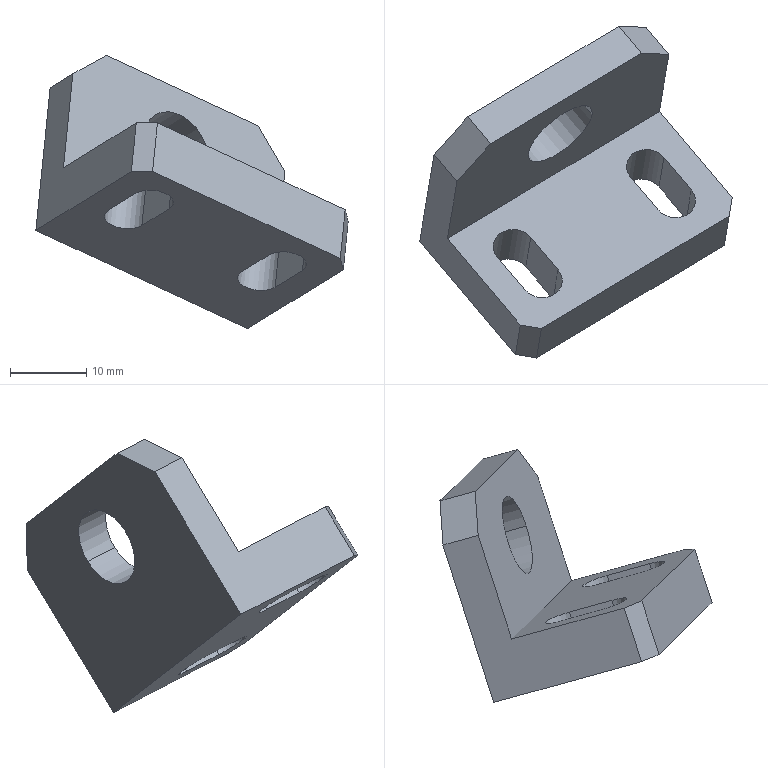Component | SolidWorks | 14AC-24-1-003-1 | 1 solid | 22 faces | box 41.09 x 43.66 x 35.95 mm | volume 8011 mm3 | plane 16 | cylinder 6 | commonest cylinder face diameters 5.5 x4 10.5 x2
build123d program:
from build123d import *

# Parameters (mm, degrees)
SKETCH1_W           = 35
SKETCH1_H           = 27
BOSS_EXTRUDE1_DEPTH = 5
SKETCH2_W           = 35
SKETCH2_H           = 7.5
BOSS_EXTRUDE2_DEPTH = 18
SKETCH3_R           = 5.25
CUT_EXTRUDE1_DEPTH  = 29.504
CHAMFER1_SIZE       = 5
CUT_EXTRUDE2_DEPTH  = 35.864
CHAMFER2_SIZE       = 2


with BuildPart() as part:
    # Sketch1 → Boss-Extrude1 (new body)
    with BuildSketch(Plane(origin=(0, 0, 0), x_dir=(0, 0, -1), z_dir=(1, 0, 0))):
        Rectangle(SKETCH1_W, SKETCH1_H)
    extrude(amount=BOSS_EXTRUDE1_DEPTH)

    # Sketch2 → Boss-Extrude2 (add)
    with BuildSketch(Plane(origin=(5, 0, 0), x_dir=(0, 0, -1), z_dir=(1, 0, 0))):
        with Locations((0, -9.75)):
            Rectangle(SKETCH2_W, SKETCH2_H)
    extrude(amount=BOSS_EXTRUDE2_DEPTH)

    # Sketch3 → Cut-Extrude1 (cut, through all)
    with BuildSketch(Plane(origin=(5, 0, 0), x_dir=(0, 0, -1), z_dir=(1, 0, 0))):
        with Locations((0, 4.5)):
            Circle(SKETCH3_R)
    extrude(amount=-CUT_EXTRUDE1_DEPTH, mode=Mode.SUBTRACT)

    # Chamfer1
    chamfer1_edges = [part.edges().sort_by_distance(p)[0] for p in [
        (2.5, 13.5, -17.5),
        (2.5, 13.5, 17.5),
    ]]
    chamfer(chamfer1_edges, length=CHAMFER1_SIZE)

    # Sketch4 → Cut-Extrude2 (cut, through all)
    with BuildSketch(Plane(origin=(0, -6, 0), x_dir=(1, 0, 0), z_dir=(0, 1, 0))):
        with BuildLine():
            Line((11, -8.25), (17, -8.25))
            ThreePointArc((17, -8.25), (19.75, -11), (17, -13.75))
            Line((17, -13.75), (11, -13.75))
            ThreePointArc((11, -13.75), (8.25, -11), (11, -8.25))
        make_face()
        with BuildLine():
            Line((11, 13.75), (17, 13.75))
            ThreePointArc((17, 13.75), (19.75, 11), (17, 8.25))
            Line((17, 8.25), (11, 8.25))
            ThreePointArc((11, 8.25), (8.25, 11), (11, 13.75))
        make_face()
    extrude(amount=-CUT_EXTRUDE2_DEPTH, mode=Mode.SUBTRACT)

    # Chamfer2
    chamfer2_edges = [part.edges().sort_by_distance(p)[0] for p in [
        (23, -9.75, -17.5),
        (23, -9.75, 17.5),
    ]]
    chamfer(chamfer2_edges, length=CHAMFER2_SIZE)


solid = part.part

# Placed as in the assembly
solid = solid.moved(Location((439.032, -206.199, -86.134), (52.359, -52.802, -8.155)))
STEP:
#1=COLOUR_RGB('',0.7922,0.8196,0.9333);
#2=FILL_AREA_STYLE_COLOUR('',#1);
#3=FILL_AREA_STYLE('',(#2));
#4=SURFACE_STYLE_FILL_AREA(#3);
#5=SURFACE_SIDE_STYLE('',(#4));
#6=SURFACE_STYLE_USAGE(.BOTH.,#5);
#7=PRESENTATION_STYLE_ASSIGNMENT((#6));
#8=CARTESIAN_POINT('',(17.135,-8.126,-3.164));
#9=VERTEX_POINT('',#8);
#10=CARTESIAN_POINT('',(17.465,-7.928,-3.316));
#11=VERTEX_POINT('',#10);
#12=CARTESIAN_POINT('',(17.3,-8.027,-3.24));
#13=DIRECTION('',(0.5985,-0.711,0.3692));
#14=DIRECTION('',(0.7966,0.4787,-0.3692));
#15=AXIS2_PLACEMENT_3D('',#12,#13,#14);
#16=CIRCLE('',#15,0.2067);
#17=EDGE_CURVE('',#9,#11,#16,.T.);
#18=ORIENTED_EDGE('',*,*,#17,.F.);
#19=CARTESIAN_POINT('',(17.253,-8.266,-3.091));
#20=VERTEX_POINT('',#19);
#21=CARTESIAN_POINT('',(17.135,-8.126,-3.164));
#22=DIRECTION('',(0.5985,-0.711,0.3692));
#23=VECTOR('',#22,39.37);
#24=LINE('',#21,#23);
#25=EDGE_CURVE('',#9,#20,#24,.T.);
#26=ORIENTED_EDGE('',*,*,#25,.T.);
#27=CARTESIAN_POINT('',(17.582,-8.068,-3.244));
#28=VERTEX_POINT('',#27);
#29=CARTESIAN_POINT('',(17.418,-8.167,-3.167));
#30=DIRECTION('',(0.5985,-0.711,0.3692));
#31=DIRECTION('',(0.7966,0.4787,-0.3692));
#32=AXIS2_PLACEMENT_3D('',#29,#30,#31);
#33=CIRCLE('',#32,0.2067);
#34=EDGE_CURVE('',#20,#28,#33,.T.);
#35=ORIENTED_EDGE('',*,*,#34,.T.);
#36=CARTESIAN_POINT('',(17.465,-7.928,-3.316));
#37=DIRECTION('',(0.5985,-0.711,0.3692));
#38=VECTOR('',#37,39.37);
#39=LINE('',#36,#38);
#40=EDGE_CURVE('',#11,#28,#39,.T.);
#41=ORIENTED_EDGE('',*,*,#40,.F.);
#42=EDGE_LOOP('',(#18,#26,#35,#41));
#43=FACE_OUTER_BOUND('',#42,.T.);
#44=CARTESIAN_POINT('',(17.3,-8.027,-3.24));
#45=DIRECTION('',(0.5985,-0.711,0.3692));
#46=DIRECTION('',(0.7966,0.4787,-0.3692));
#47=AXIS2_PLACEMENT_3D('',#44,#45,#46);
#48=CYLINDRICAL_SURFACE('',#47,0.2067);
#49=ADVANCED_FACE('',(#43),#48,.F.);
#50=CARTESIAN_POINT('',(18.308,-8.498,-3.542));
#51=VERTEX_POINT('',#50);
#52=CARTESIAN_POINT('',(17.931,-8.05,-3.774));
#53=VERTEX_POINT('',#52);
#54=CARTESIAN_POINT('',(18.355,-8.554,-3.513));
#55=DIRECTION('',(-0.5985,0.711,-0.3692));
#56=VECTOR('',#55,39.37);
#57=LINE('',#54,#56);
#58=EDGE_CURVE('',#51,#53,#57,.T.);
#59=ORIENTED_EDGE('',*,*,#58,.F.);
#60=CARTESIAN_POINT('',(18.283,-8.65,-3.793));
#61=VERTEX_POINT('',#60);
#62=CARTESIAN_POINT('',(18.374,-8.102,-2.887));
#63=DIRECTION('',(-0.08576,-0.5151,-0.8529));
#64=VECTOR('',#63,39.37);
#65=LINE('',#62,#64);
#66=EDGE_CURVE('',#51,#61,#65,.T.);
#67=ORIENTED_EDGE('',*,*,#66,.T.);
#68=CARTESIAN_POINT('',(17.788,-8.062,-4.099));
#69=VERTEX_POINT('',#68);
#70=CARTESIAN_POINT('',(17.906,-8.202,-4.026));
#71=DIRECTION('',(-0.5985,0.711,-0.3692));
#72=VECTOR('',#71,39.37);
#73=LINE('',#70,#72);
#74=EDGE_CURVE('',#61,#69,#73,.T.);
#75=ORIENTED_EDGE('',*,*,#74,.T.);
#76=CARTESIAN_POINT('',(17.862,-7.616,-3.36));
#77=VERTEX_POINT('',#76);
#78=CARTESIAN_POINT('',(17.879,-7.515,-3.192));
#79=DIRECTION('',(0.08576,0.5151,0.8529));
#80=VECTOR('',#79,39.37);
#81=LINE('',#78,#80);
#82=EDGE_CURVE('',#69,#77,#81,.T.);
#83=ORIENTED_EDGE('',*,*,#82,.T.);
#84=CARTESIAN_POINT('',(17.98,-7.756,-3.287));
#85=VERTEX_POINT('',#84);
#86=CARTESIAN_POINT('',(17.98,-7.756,-3.287));
#87=DIRECTION('',(0.5985,-0.711,0.3692));
#88=VECTOR('',#87,39.37);
#89=LINE('',#86,#88);
#90=EDGE_CURVE('',#77,#85,#89,.T.);
#91=ORIENTED_EDGE('',*,*,#90,.T.);
#92=CARTESIAN_POINT('',(17.997,-7.654,-3.12));
#93=DIRECTION('',(0.08576,0.5151,0.8529));
#94=VECTOR('',#93,39.37);
#95=LINE('',#92,#94);
#96=EDGE_CURVE('',#53,#85,#95,.T.);
#97=ORIENTED_EDGE('',*,*,#96,.F.);
#98=EDGE_LOOP('',(#59,#67,#75,#83,#91,#97));
#99=FACE_OUTER_BOUND('',#98,.T.);
#100=CARTESIAN_POINT('',(17.997,-7.654,-3.12));
#101=DIRECTION('',(-0.7966,-0.4787,0.3692));
#102=DIRECTION('',(0.5985,-0.711,0.3692));
#103=AXIS2_PLACEMENT_3D('',#100,#101,#102);
#104=PLANE('',#103);
#105=ADVANCED_FACE('',(#99),#104,.F.);
#106=CARTESIAN_POINT('',(17.84,-7.749,-3.047));
#107=VERTEX_POINT('',#106);
#108=CARTESIAN_POINT('',(17.056,-8.22,-2.683));
#109=VERTEX_POINT('',#108);
#110=CARTESIAN_POINT('',(16.899,-8.314,-2.611));
#111=DIRECTION('',(-0.7966,-0.4787,0.3692));
#112=VECTOR('',#111,39.37);
#113=LINE('',#110,#112);
#114=EDGE_CURVE('',#107,#109,#113,.T.);
#115=ORIENTED_EDGE('',*,*,#114,.F.);
#116=CARTESIAN_POINT('',(17.722,-7.609,-3.12));
#117=VERTEX_POINT('',#116);
#118=CARTESIAN_POINT('',(17.84,-7.749,-3.047));
#119=DIRECTION('',(-0.5985,0.711,-0.3692));
#120=VECTOR('',#119,39.37);
#121=LINE('',#118,#120);
#122=EDGE_CURVE('',#107,#117,#121,.T.);
#123=ORIENTED_EDGE('',*,*,#122,.T.);
#124=CARTESIAN_POINT('',(16.938,-8.08,-2.756));
#125=VERTEX_POINT('',#124);
#126=CARTESIAN_POINT('',(16.782,-8.174,-2.683));
#127=DIRECTION('',(-0.7966,-0.4787,0.3692));
#128=VECTOR('',#127,39.37);
#129=LINE('',#126,#128);
#130=EDGE_CURVE('',#117,#125,#129,.T.);
#131=ORIENTED_EDGE('',*,*,#130,.T.);
#132=CARTESIAN_POINT('',(17.056,-8.22,-2.683));
#133=DIRECTION('',(0.5985,-0.711,0.3692));
#134=VECTOR('',#133,39.37);
#135=LINE('',#132,#134);
#136=EDGE_CURVE('',#125,#109,#135,.T.);
#137=ORIENTED_EDGE('',*,*,#136,.T.);
#138=EDGE_LOOP('',(#115,#123,#131,#137));
#139=FACE_OUTER_BOUND('',#138,.T.);
#140=CARTESIAN_POINT('',(16.899,-8.314,-2.611));
#141=DIRECTION('',(-0.08576,-0.5151,-0.8529));
#142=DIRECTION('',(0.7966,0.4787,-0.3692));
#143=AXIS2_PLACEMENT_3D('',#140,#141,#142);
#144=PLANE('',#143);
#145=ADVANCED_FACE('',(#139),#144,.F.);
#146=CARTESIAN_POINT('',(17.185,-9.31,-3.285));
#147=VERTEX_POINT('',#146);
#148=CARTESIAN_POINT('',(16.69,-8.722,-3.59));
#149=VERTEX_POINT('',#148);
#150=CARTESIAN_POINT('',(16.808,-8.862,-3.517));
#151=DIRECTION('',(-0.5985,0.711,-0.3692));
#152=VECTOR('',#151,39.37);
#153=LINE('',#150,#152);
#154=EDGE_CURVE('',#147,#149,#153,.T.);
#155=ORIENTED_EDGE('',*,*,#154,.F.);
#156=CARTESIAN_POINT('',(17.21,-9.157,-3.033));
#157=VERTEX_POINT('',#156);
#158=CARTESIAN_POINT('',(17.276,-8.762,-2.378));
#159=DIRECTION('',(0.08576,0.5151,0.8529));
#160=VECTOR('',#159,39.37);
#161=LINE('',#158,#160);
#162=EDGE_CURVE('',#147,#157,#161,.T.);
#163=ORIENTED_EDGE('',*,*,#162,.T.);
#164=CARTESIAN_POINT('',(16.833,-8.71,-3.265));
#165=VERTEX_POINT('',#164);
#166=CARTESIAN_POINT('',(17.258,-9.213,-3.004));
#167=DIRECTION('',(-0.5985,0.711,-0.3692));
#168=VECTOR('',#167,39.37);
#169=LINE('',#166,#168);
#170=EDGE_CURVE('',#157,#165,#169,.T.);
#171=ORIENTED_EDGE('',*,*,#170,.T.);
#172=CARTESIAN_POINT('',(16.882,-8.416,-2.779));
#173=VERTEX_POINT('',#172);
#174=CARTESIAN_POINT('',(16.899,-8.314,-2.611));
#175=DIRECTION('',(-0.08576,-0.5151,-0.8529));
#176=VECTOR('',#175,39.37);
#177=LINE('',#174,#176);
#178=EDGE_CURVE('',#173,#165,#177,.T.);
#179=ORIENTED_EDGE('',*,*,#178,.F.);
#180=CARTESIAN_POINT('',(16.765,-8.276,-2.851));
#181=VERTEX_POINT('',#180);
#182=CARTESIAN_POINT('',(16.882,-8.416,-2.779));
#183=DIRECTION('',(-0.5985,0.711,-0.3692));
#184=VECTOR('',#183,39.37);
#185=LINE('',#182,#184);
#186=EDGE_CURVE('',#173,#181,#185,.T.);
#187=ORIENTED_EDGE('',*,*,#186,.T.);
#188=CARTESIAN_POINT('',(16.782,-8.174,-2.683));
#189=DIRECTION('',(-0.08576,-0.5151,-0.8529));
#190=VECTOR('',#189,39.37);
#191=LINE('',#188,#190);
#192=EDGE_CURVE('',#181,#149,#191,.T.);
#193=ORIENTED_EDGE('',*,*,#192,.T.);
#194=EDGE_LOOP('',(#155,#163,#171,#179,#187,#193));
#195=FACE_OUTER_BOUND('',#194,.T.);
#196=CARTESIAN_POINT('',(16.899,-8.314,-2.611));
#197=DIRECTION('',(0.7966,0.4787,-0.3692));
#198=DIRECTION('',(0.08576,0.5151,0.8529));
#199=AXIS2_PLACEMENT_3D('',#196,#197,#198);
#200=PLANE('',#199);
#201=ADVANCED_FACE('',(#195),#200,.F.);
#202=CARTESIAN_POINT('',(18.071,-8.609,-3.797));
#203=VERTEX_POINT('',#202);
#204=CARTESIAN_POINT('',(17.93,-8.441,-3.884));
#205=VERTEX_POINT('',#204);
#206=CARTESIAN_POINT('',(17.93,-8.441,-3.884));
#207=DIRECTION('',(-0.5985,0.711,-0.3692));
#208=VECTOR('',#207,39.37);
#209=LINE('',#206,#208);
#210=EDGE_CURVE('',#203,#205,#209,.T.);
#211=ORIENTED_EDGE('',*,*,#210,.T.);
#212=CARTESIAN_POINT('',(17.757,-8.544,-3.804));
#213=VERTEX_POINT('',#212);
#214=CARTESIAN_POINT('',(17.843,-8.492,-3.844));
#215=DIRECTION('',(0.08576,0.5151,0.8529));
#216=DIRECTION('',(-0.7966,-0.4787,0.3692));
#217=AXIS2_PLACEMENT_3D('',#214,#215,#216);
#218=CIRCLE('',#217,0.1083);
#219=EDGE_CURVE('',#205,#213,#218,.T.);
#220=ORIENTED_EDGE('',*,*,#219,.T.);
#221=CARTESIAN_POINT('',(17.898,-8.712,-3.717));
#222=VERTEX_POINT('',#221);
#223=CARTESIAN_POINT('',(17.757,-8.544,-3.804));
#224=DIRECTION('',(0.5985,-0.711,0.3692));
#225=VECTOR('',#224,39.37);
#226=LINE('',#223,#225);
#227=EDGE_CURVE('',#213,#222,#226,.T.);
#228=ORIENTED_EDGE('',*,*,#227,.T.);
#229=CARTESIAN_POINT('',(17.985,-8.66,-3.757));
#230=DIRECTION('',(0.08576,0.5151,0.8529));
#231=DIRECTION('',(-0.7966,-0.4787,0.3692));
#232=AXIS2_PLACEMENT_3D('',#229,#230,#231);
#233=CIRCLE('',#232,0.1083);
#234=EDGE_CURVE('',#222,#203,#233,.T.);
#235=ORIENTED_EDGE('',*,*,#234,.T.);
#236=EDGE_LOOP('',(#211,#220,#228,#235));
#237=FACE_BOUND('',#236,.T.);
#238=CARTESIAN_POINT('',(17.381,-9.023,-3.477));
#239=VERTEX_POINT('',#238);
#240=CARTESIAN_POINT('',(17.24,-8.855,-3.565));
#241=VERTEX_POINT('',#240);
#242=CARTESIAN_POINT('',(17.24,-8.855,-3.565));
#243=DIRECTION('',(-0.5985,0.711,-0.3692));
#244=VECTOR('',#243,39.37);
#245=LINE('',#242,#244);
#246=EDGE_CURVE('',#239,#241,#245,.T.);
#247=ORIENTED_EDGE('',*,*,#246,.T.);
#248=CARTESIAN_POINT('',(17.067,-8.959,-3.485));
#249=VERTEX_POINT('',#248);
#250=CARTESIAN_POINT('',(17.153,-8.907,-3.525));
#251=DIRECTION('',(0.08576,0.5151,0.8529));
#252=DIRECTION('',(-0.7966,-0.4787,0.3692));
#253=AXIS2_PLACEMENT_3D('',#250,#251,#252);
#254=CIRCLE('',#253,0.1083);
#255=EDGE_CURVE('',#241,#249,#254,.T.);
#256=ORIENTED_EDGE('',*,*,#255,.T.);
#257=CARTESIAN_POINT('',(17.208,-9.127,-3.397));
#258=VERTEX_POINT('',#257);
#259=CARTESIAN_POINT('',(17.067,-8.959,-3.485));
#260=DIRECTION('',(0.5985,-0.711,0.3692));
#261=VECTOR('',#260,39.37);
#262=LINE('',#259,#261);
#263=EDGE_CURVE('',#249,#258,#262,.T.);
#264=ORIENTED_EDGE('',*,*,#263,.T.);
#265=CARTESIAN_POINT('',(17.295,-9.075,-3.437));
#266=DIRECTION('',(0.08576,0.5151,0.8529));
#267=DIRECTION('',(-0.7966,-0.4787,0.3692));
#268=AXIS2_PLACEMENT_3D('',#265,#266,#267);
#269=CIRCLE('',#268,0.1083);
#270=EDGE_CURVE('',#258,#239,#269,.T.);
#271=ORIENTED_EDGE('',*,*,#270,.T.);
#272=EDGE_LOOP('',(#247,#256,#264,#271));
#273=FACE_BOUND('',#272,.T.);
#274=ORIENTED_EDGE('',*,*,#74,.F.);
#275=CARTESIAN_POINT('',(18.267,-8.744,-3.735));
#276=VERTEX_POINT('',#275);
#277=CARTESIAN_POINT('',(18.267,-8.744,-3.735));
#278=DIRECTION('',(-0.1401,-0.8413,0.5222));
#279=VECTOR('',#278,39.37);
#280=LINE('',#277,#279);
#281=EDGE_CURVE('',#61,#276,#280,.T.);
#282=ORIENTED_EDGE('',*,*,#281,.T.);
#283=CARTESIAN_POINT('',(17.295,-9.328,-3.285));
#284=VERTEX_POINT('',#283);
#285=CARTESIAN_POINT('',(17.232,-9.365,-3.256));
#286=DIRECTION('',(0.7966,0.4787,-0.3692));
#287=VECTOR('',#286,39.37);
#288=LINE('',#285,#287);
#289=EDGE_CURVE('',#284,#276,#288,.T.);
#290=ORIENTED_EDGE('',*,*,#289,.F.);
#291=CARTESIAN_POINT('',(17.295,-9.328,-3.285));
#292=DIRECTION('',(-0.9864,0.1642,-0.));
#293=VECTOR('',#292,39.37);
#294=LINE('',#291,#293);
#295=EDGE_CURVE('',#284,#147,#294,.T.);
#296=ORIENTED_EDGE('',*,*,#295,.T.);
#297=ORIENTED_EDGE('',*,*,#154,.T.);
#298=CARTESIAN_POINT('',(16.69,-8.722,-3.59));
#299=DIRECTION('',(0.7966,0.4787,-0.3692));
#300=VECTOR('',#299,39.37);
#301=LINE('',#298,#300);
#302=EDGE_CURVE('',#149,#69,#301,.T.);
#303=ORIENTED_EDGE('',*,*,#302,.T.);
#304=EDGE_LOOP('',(#274,#282,#290,#296,#297,#303));
#305=FACE_OUTER_BOUND('',#304,.T.);
#306=CARTESIAN_POINT('',(16.808,-8.862,-3.517));
#307=DIRECTION('',(0.08576,0.5151,0.8529));
#308=DIRECTION('',(-0.7966,-0.4787,0.3692));
#309=AXIS2_PLACEMENT_3D('',#306,#307,#308);
#310=PLANE('',#309);
#311=ADVANCED_FACE('',(#237,#273,#305),#310,.F.);
#312=CARTESIAN_POINT('',(17.418,-8.167,-3.167));
#313=DIRECTION('',(0.5985,-0.711,0.3692));
#314=DIRECTION('',(0.7966,0.4787,-0.3692));
#315=AXIS2_PLACEMENT_3D('',#312,#313,#314);
#316=CIRCLE('',#315,0.2067);
#317=EDGE_CURVE('',#28,#20,#316,.T.);
#318=ORIENTED_EDGE('',*,*,#317,.F.);
#319=ORIENTED_EDGE('',*,*,#34,.F.);
#320=EDGE_LOOP('',(#318,#319));
#321=FACE_BOUND('',#320,.T.);
#322=ORIENTED_EDGE('',*,*,#96,.T.);
#323=CARTESIAN_POINT('',(17.854,-7.749,-3.071));
#324=DIRECTION('',(-0.5026,0.0257,0.8641));
#325=VECTOR('',#324,39.37);
#326=LINE('',#323,#325);
#327=EDGE_CURVE('',#85,#107,#326,.T.);
#328=ORIENTED_EDGE('',*,*,#327,.T.);
#329=ORIENTED_EDGE('',*,*,#114,.T.);
#330=CARTESIAN_POINT('',(17.039,-8.239,-2.693));
#331=DIRECTION('',(-0.6239,-0.7027,-0.342));
#332=VECTOR('',#331,39.37);
#333=LINE('',#330,#332);
#334=EDGE_CURVE('',#109,#173,#333,.T.);
#335=ORIENTED_EDGE('',*,*,#334,.T.);
#336=ORIENTED_EDGE('',*,*,#178,.T.);
#337=CARTESIAN_POINT('',(16.833,-8.71,-3.265));
#338=DIRECTION('',(-0.7966,-0.4787,0.3692));
#339=VECTOR('',#338,39.37);
#340=LINE('',#337,#339);
#341=EDGE_CURVE('',#53,#165,#340,.T.);
#342=ORIENTED_EDGE('',*,*,#341,.F.);
#343=EDGE_LOOP('',(#322,#328,#329,#335,#336,#342));
#344=FACE_OUTER_BOUND('',#343,.T.);
#345=CARTESIAN_POINT('',(17.403,-8.258,-3.318));
#346=DIRECTION('',(0.5985,-0.711,0.3692));
#347=DIRECTION('',(0.7966,0.4787,-0.3692));
#348=AXIS2_PLACEMENT_3D('',#345,#346,#347);
#349=PLANE('',#348);
#350=ADVANCED_FACE('',(#321,#344),#349,.T.);
#351=CARTESIAN_POINT('',(17.3,-8.027,-3.24));
#352=DIRECTION('',(0.5985,-0.711,0.3692));
#353=DIRECTION('',(0.7966,0.4787,-0.3692));
#354=AXIS2_PLACEMENT_3D('',#351,#352,#353);
#355=CIRCLE('',#354,0.2067);
#356=EDGE_CURVE('',#11,#9,#355,.T.);
#357=ORIENTED_EDGE('',*,*,#356,.T.);
#358=ORIENTED_EDGE('',*,*,#17,.T.);
#359=EDGE_LOOP('',(#357,#358));
#360=FACE_BOUND('',#359,.T.);
#361=ORIENTED_EDGE('',*,*,#130,.F.);
#362=CARTESIAN_POINT('',(17.722,-7.609,-3.12));
#363=DIRECTION('',(0.5026,-0.0257,-0.8641));
#364=VECTOR('',#363,39.37);
#365=LINE('',#362,#364);
#366=EDGE_CURVE('',#117,#77,#365,.T.);
#367=ORIENTED_EDGE('',*,*,#366,.T.);
#368=ORIENTED_EDGE('',*,*,#82,.F.);
#369=ORIENTED_EDGE('',*,*,#302,.F.);
#370=ORIENTED_EDGE('',*,*,#192,.F.);
#371=CARTESIAN_POINT('',(16.765,-8.276,-2.851));
#372=DIRECTION('',(0.6239,0.7027,0.342));
#373=VECTOR('',#372,39.37);
#374=LINE('',#371,#373);
#375=EDGE_CURVE('',#181,#125,#374,.T.);
#376=ORIENTED_EDGE('',*,*,#375,.T.);
#377=EDGE_LOOP('',(#361,#367,#368,#369,#370,#376));
#378=FACE_OUTER_BOUND('',#377,.T.);
#379=CARTESIAN_POINT('',(17.285,-8.118,-3.391));
#380=DIRECTION('',(0.5985,-0.711,0.3692));
#381=DIRECTION('',(0.7966,0.4787,-0.3692));
#382=AXIS2_PLACEMENT_3D('',#379,#380,#381);
#383=PLANE('',#382);
#384=ADVANCED_FACE('',(#360,#378),#383,.F.);
#385=CARTESIAN_POINT('',(17.782,-8.392,-3.553));
#386=VERTEX_POINT('',#385);
#387=CARTESIAN_POINT('',(17.924,-8.56,-3.465));
#388=VERTEX_POINT('',#387);
#389=CARTESIAN_POINT('',(17.782,-8.392,-3.553));
#390=DIRECTION('',(0.5985,-0.711,0.3692));
#391=VECTOR('',#390,39.37);
#392=LINE('',#389,#391);
#393=EDGE_CURVE('',#386,#388,#392,.T.);
#394=ORIENTED_EDGE('',*,*,#393,.F.);
#395=CARTESIAN_POINT('',(17.955,-8.289,-3.633));
#396=VERTEX_POINT('',#395);
#397=CARTESIAN_POINT('',(17.869,-8.34,-3.593));
#398=DIRECTION('',(0.08576,0.5151,0.8529));
#399=DIRECTION('',(-0.7966,-0.4787,0.3692));
#400=AXIS2_PLACEMENT_3D('',#397,#398,#399);
#401=CIRCLE('',#400,0.1083);
#402=EDGE_CURVE('',#396,#386,#401,.T.);
#403=ORIENTED_EDGE('',*,*,#402,.F.);
#404=CARTESIAN_POINT('',(18.096,-8.456,-3.545));
#405=VERTEX_POINT('',#404);
#406=CARTESIAN_POINT('',(17.955,-8.289,-3.633));
#407=DIRECTION('',(-0.5985,0.711,-0.3692));
#408=VECTOR('',#407,39.37);
#409=LINE('',#406,#408);
#410=EDGE_CURVE('',#405,#396,#409,.T.);
#411=ORIENTED_EDGE('',*,*,#410,.F.);
#412=CARTESIAN_POINT('',(18.01,-8.508,-3.505));
#413=DIRECTION('',(0.08576,0.5151,0.8529));
#414=DIRECTION('',(-0.7966,-0.4787,0.3692));
#415=AXIS2_PLACEMENT_3D('',#412,#413,#414);
#416=CIRCLE('',#415,0.1083);
#417=EDGE_CURVE('',#388,#405,#416,.T.);
#418=ORIENTED_EDGE('',*,*,#417,.F.);
#419=EDGE_LOOP('',(#394,#403,#411,#418));
#420=FACE_BOUND('',#419,.T.);
#421=CARTESIAN_POINT('',(17.092,-8.807,-3.233));
#422=VERTEX_POINT('',#421);
#423=CARTESIAN_POINT('',(17.234,-8.975,-3.146));
#424=VERTEX_POINT('',#423);
#425=CARTESIAN_POINT('',(17.092,-8.807,-3.233));
#426=DIRECTION('',(0.5985,-0.711,0.3692));
#427=VECTOR('',#426,39.37);
#428=LINE('',#425,#427);
#429=EDGE_CURVE('',#422,#424,#428,.T.);
#430=ORIENTED_EDGE('',*,*,#429,.F.);
#431=CARTESIAN_POINT('',(17.265,-8.703,-3.313));
#432=VERTEX_POINT('',#431);
#433=CARTESIAN_POINT('',(17.179,-8.755,-3.273));
#434=DIRECTION('',(0.08576,0.5151,0.8529));
#435=DIRECTION('',(-0.7966,-0.4787,0.3692));
#436=AXIS2_PLACEMENT_3D('',#433,#434,#435);
#437=CIRCLE('',#436,0.1083);
#438=EDGE_CURVE('',#432,#422,#437,.T.);
#439=ORIENTED_EDGE('',*,*,#438,.F.);
#440=CARTESIAN_POINT('',(17.406,-8.871,-3.226));
#441=VERTEX_POINT('',#440);
#442=CARTESIAN_POINT('',(17.265,-8.703,-3.313));
#443=DIRECTION('',(-0.5985,0.711,-0.3692));
#444=VECTOR('',#443,39.37);
#445=LINE('',#442,#444);
#446=EDGE_CURVE('',#441,#432,#445,.T.);
#447=ORIENTED_EDGE('',*,*,#446,.F.);
#448=CARTESIAN_POINT('',(17.32,-8.923,-3.186));
#449=DIRECTION('',(0.08576,0.5151,0.8529));
#450=DIRECTION('',(-0.7966,-0.4787,0.3692));
#451=AXIS2_PLACEMENT_3D('',#448,#449,#450);
#452=CIRCLE('',#451,0.1083);
#453=EDGE_CURVE('',#424,#441,#452,.T.);
#454=ORIENTED_EDGE('',*,*,#453,.F.);
#455=EDGE_LOOP('',(#430,#439,#447,#454));
#456=FACE_BOUND('',#455,.T.);
#457=CARTESIAN_POINT('',(18.292,-8.591,-3.484));
#458=VERTEX_POINT('',#457);
#459=CARTESIAN_POINT('',(17.32,-9.176,-3.033));
#460=VERTEX_POINT('',#459);
#461=CARTESIAN_POINT('',(17.258,-9.213,-3.004));
#462=DIRECTION('',(-0.7966,-0.4787,0.3692));
#463=VECTOR('',#462,39.37);
#464=LINE('',#461,#463);
#465=EDGE_CURVE('',#458,#460,#464,.T.);
#466=ORIENTED_EDGE('',*,*,#465,.F.);
#467=CARTESIAN_POINT('',(18.292,-8.591,-3.484));
#468=DIRECTION('',(0.1401,0.8413,-0.5222));
#469=VECTOR('',#468,39.37);
#470=LINE('',#467,#469);
#471=EDGE_CURVE('',#458,#51,#470,.T.);
#472=ORIENTED_EDGE('',*,*,#471,.T.);
#473=ORIENTED_EDGE('',*,*,#58,.T.);
#474=ORIENTED_EDGE('',*,*,#341,.T.);
#475=ORIENTED_EDGE('',*,*,#170,.F.);
#476=CARTESIAN_POINT('',(17.32,-9.176,-3.033));
#477=DIRECTION('',(0.9864,-0.1642,0.));
#478=VECTOR('',#477,39.37);
#479=LINE('',#476,#478);
#480=EDGE_CURVE('',#157,#460,#479,.T.);
#481=ORIENTED_EDGE('',*,*,#480,.T.);
#482=EDGE_LOOP('',(#466,#472,#473,#474,#475,#481));
#483=FACE_OUTER_BOUND('',#482,.T.);
#484=CARTESIAN_POINT('',(17.258,-9.213,-3.004));
#485=DIRECTION('',(-0.08576,-0.5151,-0.8529));
#486=DIRECTION('',(0.7966,0.4787,-0.3692));
#487=AXIS2_PLACEMENT_3D('',#484,#485,#486);
#488=PLANE('',#487);
#489=ADVANCED_FACE('',(#420,#456,#483),#488,.F.);
#490=ORIENTED_EDGE('',*,*,#289,.T.);
#491=CARTESIAN_POINT('',(18.313,-8.47,-3.282));
#492=DIRECTION('',(0.08576,0.5151,0.8529));
#493=VECTOR('',#492,39.37);
#494=LINE('',#491,#493);
#495=EDGE_CURVE('',#276,#458,#494,.T.);
#496=ORIENTED_EDGE('',*,*,#495,.T.);
#497=ORIENTED_EDGE('',*,*,#465,.T.);
#498=CARTESIAN_POINT('',(17.341,-9.054,-2.831));
#499=DIRECTION('',(-0.08576,-0.5151,-0.8529));
#500=VECTOR('',#499,39.37);
#501=LINE('',#498,#500);
#502=EDGE_CURVE('',#460,#284,#501,.T.);
#503=ORIENTED_EDGE('',*,*,#502,.T.);
#504=EDGE_LOOP('',(#490,#496,#497,#503));
#505=FACE_OUTER_BOUND('',#504,.T.);
#506=CARTESIAN_POINT('',(17.827,-8.762,-3.057));
#507=DIRECTION('',(-0.5985,0.711,-0.3692));
#508=DIRECTION('',(-0.7966,-0.4787,0.3692));
#509=AXIS2_PLACEMENT_3D('',#506,#507,#508);
#510=PLANE('',#509);
#511=ADVANCED_FACE('',(#505),#510,.F.);
#512=ORIENTED_EDGE('',*,*,#25,.F.);
#513=ORIENTED_EDGE('',*,*,#356,.F.);
#514=ORIENTED_EDGE('',*,*,#40,.T.);
#515=ORIENTED_EDGE('',*,*,#317,.T.);
#516=EDGE_LOOP('',(#512,#513,#514,#515));
#517=FACE_OUTER_BOUND('',#516,.T.);
#518=CARTESIAN_POINT('',(17.3,-8.027,-3.24));
#519=DIRECTION('',(0.5985,-0.711,0.3692));
#520=DIRECTION('',(0.7966,0.4787,-0.3692));
#521=AXIS2_PLACEMENT_3D('',#518,#519,#520);
#522=CYLINDRICAL_SURFACE('',#521,0.2067);
#523=ADVANCED_FACE('',(#517),#522,.F.);
#524=ORIENTED_EDGE('',*,*,#327,.F.);
#525=ORIENTED_EDGE('',*,*,#90,.F.);
#526=ORIENTED_EDGE('',*,*,#366,.F.);
#527=ORIENTED_EDGE('',*,*,#122,.F.);
#528=EDGE_LOOP('',(#524,#525,#526,#527));
#529=FACE_OUTER_BOUND('',#528,.T.);
#530=CARTESIAN_POINT('',(17.84,-7.749,-3.047));
#531=DIRECTION('',(-0.6239,-0.7027,-0.342));
#532=DIRECTION('',(-0.5985,0.711,-0.3692));
#533=AXIS2_PLACEMENT_3D('',#530,#531,#532);
#534=PLANE('',#533);
#535=ADVANCED_FACE('',(#529),#534,.F.);
#536=ORIENTED_EDGE('',*,*,#334,.F.);
#537=ORIENTED_EDGE('',*,*,#136,.F.);
#538=ORIENTED_EDGE('',*,*,#375,.F.);
#539=ORIENTED_EDGE('',*,*,#186,.F.);
#540=EDGE_LOOP('',(#536,#537,#538,#539));
#541=FACE_OUTER_BOUND('',#540,.T.);
#542=CARTESIAN_POINT('',(16.882,-8.416,-2.779));
#543=DIRECTION('',(0.5026,-0.0257,-0.8641));
#544=DIRECTION('',(-0.5985,0.711,-0.3692));
#545=AXIS2_PLACEMENT_3D('',#542,#543,#544);
#546=PLANE('',#545);
#547=ADVANCED_FACE('',(#541),#546,.F.);
#548=ORIENTED_EDGE('',*,*,#438,.T.);
#549=CARTESIAN_POINT('',(17.067,-8.959,-3.485));
#550=DIRECTION('',(0.08576,0.5151,0.8529));
#551=VECTOR('',#550,39.37);
#552=LINE('',#549,#551);
#553=EDGE_CURVE('',#249,#422,#552,.T.);
#554=ORIENTED_EDGE('',*,*,#553,.F.);
#555=ORIENTED_EDGE('',*,*,#255,.F.);
#556=CARTESIAN_POINT('',(17.24,-8.855,-3.565));
#557=DIRECTION('',(0.08576,0.5151,0.8529));
#558=VECTOR('',#557,39.37);
#559=LINE('',#556,#558);
#560=EDGE_CURVE('',#241,#432,#559,.T.);
#561=ORIENTED_EDGE('',*,*,#560,.T.);
#562=EDGE_LOOP('',(#548,#554,#555,#561));
#563=FACE_OUTER_BOUND('',#562,.T.);
#564=CARTESIAN_POINT('',(17.153,-8.907,-3.525));
#565=DIRECTION('',(0.08576,0.5151,0.8529));
#566=DIRECTION('',(-0.7966,-0.4787,0.3692));
#567=AXIS2_PLACEMENT_3D('',#564,#565,#566);
#568=CYLINDRICAL_SURFACE('',#567,0.1083);
#569=ADVANCED_FACE('',(#563),#568,.F.);
#570=ORIENTED_EDGE('',*,*,#446,.T.);
#571=ORIENTED_EDGE('',*,*,#560,.F.);
#572=ORIENTED_EDGE('',*,*,#246,.F.);
#573=CARTESIAN_POINT('',(17.381,-9.023,-3.477));
#574=DIRECTION('',(0.08576,0.5151,0.8529));
#575=VECTOR('',#574,39.37);
#576=LINE('',#573,#575);
#577=EDGE_CURVE('',#239,#441,#576,.T.);
#578=ORIENTED_EDGE('',*,*,#577,.T.);
#579=EDGE_LOOP('',(#570,#571,#572,#578));
#580=FACE_OUTER_BOUND('',#579,.T.);
#581=CARTESIAN_POINT('',(17.24,-8.855,-3.565));
#582=DIRECTION('',(0.7966,0.4787,-0.3692));
#583=DIRECTION('',(-0.5985,0.711,-0.3692));
#584=AXIS2_PLACEMENT_3D('',#581,#582,#583);
#585=PLANE('',#584);
#586=ADVANCED_FACE('',(#580),#585,.F.);
#587=ORIENTED_EDGE('',*,*,#453,.T.);
#588=ORIENTED_EDGE('',*,*,#577,.F.);
#589=ORIENTED_EDGE('',*,*,#270,.F.);
#590=CARTESIAN_POINT('',(17.208,-9.127,-3.397));
#591=DIRECTION('',(0.08576,0.5151,0.8529));
#592=VECTOR('',#591,39.37);
#593=LINE('',#590,#592);
#594=EDGE_CURVE('',#258,#424,#593,.T.);
#595=ORIENTED_EDGE('',*,*,#594,.T.);
#596=EDGE_LOOP('',(#587,#588,#589,#595));
#597=FACE_OUTER_BOUND('',#596,.T.);
#598=CARTESIAN_POINT('',(17.295,-9.075,-3.437));
#599=DIRECTION('',(0.08576,0.5151,0.8529));
#600=DIRECTION('',(-0.7966,-0.4787,0.3692));
#601=AXIS2_PLACEMENT_3D('',#598,#599,#600);
#602=CYLINDRICAL_SURFACE('',#601,0.1083);
#603=ADVANCED_FACE('',(#597),#602,.F.);
#604=ORIENTED_EDGE('',*,*,#429,.T.);
#605=ORIENTED_EDGE('',*,*,#594,.F.);
#606=ORIENTED_EDGE('',*,*,#263,.F.);
#607=ORIENTED_EDGE('',*,*,#553,.T.);
#608=EDGE_LOOP('',(#604,#605,#606,#607));
#609=FACE_OUTER_BOUND('',#608,.T.);
#610=CARTESIAN_POINT('',(17.067,-8.959,-3.485));
#611=DIRECTION('',(-0.7966,-0.4787,0.3692));
#612=DIRECTION('',(0.5985,-0.711,0.3692));
#613=AXIS2_PLACEMENT_3D('',#610,#611,#612);
#614=PLANE('',#613);
#615=ADVANCED_FACE('',(#609),#614,.F.);
#616=ORIENTED_EDGE('',*,*,#402,.T.);
#617=CARTESIAN_POINT('',(17.757,-8.544,-3.804));
#618=DIRECTION('',(0.08576,0.5151,0.8529));
#619=VECTOR('',#618,39.37);
#620=LINE('',#617,#619);
#621=EDGE_CURVE('',#213,#386,#620,.T.);
#622=ORIENTED_EDGE('',*,*,#621,.F.);
#623=ORIENTED_EDGE('',*,*,#219,.F.);
#624=CARTESIAN_POINT('',(17.93,-8.441,-3.884));
#625=DIRECTION('',(0.08576,0.5151,0.8529));
#626=VECTOR('',#625,39.37);
#627=LINE('',#624,#626);
#628=EDGE_CURVE('',#205,#396,#627,.T.);
#629=ORIENTED_EDGE('',*,*,#628,.T.);
#630=EDGE_LOOP('',(#616,#622,#623,#629));
#631=FACE_OUTER_BOUND('',#630,.T.);
#632=CARTESIAN_POINT('',(17.843,-8.492,-3.844));
#633=DIRECTION('',(0.08576,0.5151,0.8529));
#634=DIRECTION('',(-0.7966,-0.4787,0.3692));
#635=AXIS2_PLACEMENT_3D('',#632,#633,#634);
#636=CYLINDRICAL_SURFACE('',#635,0.1083);
#637=ADVANCED_FACE('',(#631),#636,.F.);
#638=ORIENTED_EDGE('',*,*,#410,.T.);
#639=ORIENTED_EDGE('',*,*,#628,.F.);
#640=ORIENTED_EDGE('',*,*,#210,.F.);
#641=CARTESIAN_POINT('',(18.071,-8.609,-3.797));
#642=DIRECTION('',(0.08576,0.5151,0.8529));
#643=VECTOR('',#642,39.37);
#644=LINE('',#641,#643);
#645=EDGE_CURVE('',#203,#405,#644,.T.);
#646=ORIENTED_EDGE('',*,*,#645,.T.);
#647=EDGE_LOOP('',(#638,#639,#640,#646));
#648=FACE_OUTER_BOUND('',#647,.T.);
#649=CARTESIAN_POINT('',(17.93,-8.441,-3.884));
#650=DIRECTION('',(0.7966,0.4787,-0.3692));
#651=DIRECTION('',(-0.5985,0.711,-0.3692));
#652=AXIS2_PLACEMENT_3D('',#649,#650,#651);
#653=PLANE('',#652);
#654=ADVANCED_FACE('',(#648),#653,.F.);
#655=ORIENTED_EDGE('',*,*,#417,.T.);
#656=ORIENTED_EDGE('',*,*,#645,.F.);
#657=ORIENTED_EDGE('',*,*,#234,.F.);
#658=CARTESIAN_POINT('',(17.898,-8.712,-3.717));
#659=DIRECTION('',(0.08576,0.5151,0.8529));
#660=VECTOR('',#659,39.37);
#661=LINE('',#658,#660);
#662=EDGE_CURVE('',#222,#388,#661,.T.);
#663=ORIENTED_EDGE('',*,*,#662,.T.);
#664=EDGE_LOOP('',(#655,#656,#657,#663));
#665=FACE_OUTER_BOUND('',#664,.T.);
#666=CARTESIAN_POINT('',(17.985,-8.66,-3.757));
#667=DIRECTION('',(0.08576,0.5151,0.8529));
#668=DIRECTION('',(-0.7966,-0.4787,0.3692));
#669=AXIS2_PLACEMENT_3D('',#666,#667,#668);
#670=CYLINDRICAL_SURFACE('',#669,0.1083);
#671=ADVANCED_FACE('',(#665),#670,.F.);
#672=ORIENTED_EDGE('',*,*,#393,.T.);
#673=ORIENTED_EDGE('',*,*,#662,.F.);
#674=ORIENTED_EDGE('',*,*,#227,.F.);
#675=ORIENTED_EDGE('',*,*,#621,.T.);
#676=EDGE_LOOP('',(#672,#673,#674,#675));
#677=FACE_OUTER_BOUND('',#676,.T.);
#678=CARTESIAN_POINT('',(17.757,-8.544,-3.804));
#679=DIRECTION('',(-0.7966,-0.4787,0.3692));
#680=DIRECTION('',(0.5985,-0.711,0.3692));
#681=AXIS2_PLACEMENT_3D('',#678,#679,#680);
#682=PLANE('',#681);
#683=ADVANCED_FACE('',(#677),#682,.F.);
#684=ORIENTED_EDGE('',*,*,#281,.F.);
#685=ORIENTED_EDGE('',*,*,#66,.F.);
#686=ORIENTED_EDGE('',*,*,#471,.F.);
#687=ORIENTED_EDGE('',*,*,#495,.F.);
#688=EDGE_LOOP('',(#684,#685,#686,#687));
#689=FACE_OUTER_BOUND('',#688,.T.);
#690=CARTESIAN_POINT('',(18.313,-8.47,-3.282));
#691=DIRECTION('',(-0.9864,0.1642,0.));
#692=DIRECTION('',(0.08576,0.5151,0.8529));
#693=AXIS2_PLACEMENT_3D('',#690,#691,#692);
#694=PLANE('',#693);
#695=ADVANCED_FACE('',(#689),#694,.F.);
#696=ORIENTED_EDGE('',*,*,#480,.F.);
#697=ORIENTED_EDGE('',*,*,#162,.F.);
#698=ORIENTED_EDGE('',*,*,#295,.F.);
#699=ORIENTED_EDGE('',*,*,#502,.F.);
#700=EDGE_LOOP('',(#696,#697,#698,#699));
#701=FACE_OUTER_BOUND('',#700,.T.);
#702=CARTESIAN_POINT('',(17.341,-9.054,-2.831));
#703=DIRECTION('',(0.1401,0.8413,-0.5222));
#704=DIRECTION('',(-0.08576,-0.5151,-0.8529));
#705=AXIS2_PLACEMENT_3D('',#702,#703,#704);
#706=PLANE('',#705);
#707=ADVANCED_FACE('',(#701),#706,.F.);
#708=CLOSED_SHELL('',(#49,#105,#145,#201,#311,#350,#384,#489,#511,#523,#535,#547,#569,#586,#603,#615,#637,#654,#671,#683,#695,#707));
#709=MANIFOLD_SOLID_BREP('',#708);
#710=STYLED_ITEM('',(#7),#709);
#711=PRESENTATION_LAYER_ASSIGNMENT('','',(#710));
#712=(LENGTH_UNIT()NAMED_UNIT(*)SI_UNIT($,.METRE.));
#713=LENGTH_MEASURE_WITH_UNIT(LENGTH_MEASURE(0.0254),#712);
#714=DIMENSIONAL_EXPONENTS(1.,0.,0.,0.,0.,0.,0.);
#715=(CONVERSION_BASED_UNIT('',#713)LENGTH_UNIT()NAMED_UNIT(#714));
#716=UNCERTAINTY_MEASURE_WITH_UNIT(LENGTH_MEASURE(0.00001),#715,'','');
#717=(NAMED_UNIT(*)PLANE_ANGLE_UNIT()SI_UNIT($,.RADIAN.));
#718=(NAMED_UNIT(*)SI_UNIT($,.STERADIAN.)SOLID_ANGLE_UNIT());
#719=(GEOMETRIC_REPRESENTATION_CONTEXT(3)GLOBAL_UNCERTAINTY_ASSIGNED_CONTEXT((#716))GLOBAL_UNIT_ASSIGNED_CONTEXT((#715,#717,#718))REPRESENTATION_CONTEXT('',''));
#720=MECHANICAL_DESIGN_GEOMETRIC_PRESENTATION_REPRESENTATION('',(#710),#719);
#721=CARTESIAN_POINT('',(0.,0.,0.));
#722=DIRECTION('',(0.,0.,1.));
#723=DIRECTION('',(1.,0.,0.));
#724=AXIS2_PLACEMENT_3D('',#721,#722,#723);
#725=(LENGTH_UNIT()NAMED_UNIT(*)SI_UNIT($,.METRE.));
#726=LENGTH_MEASURE_WITH_UNIT(LENGTH_MEASURE(0.0254),#725);
#727=DIMENSIONAL_EXPONENTS(1.,0.,0.,0.,0.,0.,0.);
#728=(CONVERSION_BASED_UNIT('',#726)LENGTH_UNIT()NAMED_UNIT(#727));
#729=UNCERTAINTY_MEASURE_WITH_UNIT(LENGTH_MEASURE(0.00001),#728,'','');
#730=(NAMED_UNIT(*)PLANE_ANGLE_UNIT()SI_UNIT($,.RADIAN.));
#731=(NAMED_UNIT(*)SI_UNIT($,.STERADIAN.)SOLID_ANGLE_UNIT());
#732=(GEOMETRIC_REPRESENTATION_CONTEXT(3)GLOBAL_UNCERTAINTY_ASSIGNED_CONTEXT((#729))GLOBAL_UNIT_ASSIGNED_CONTEXT((#728,#730,#731))REPRESENTATION_CONTEXT('',''));
#733=ADVANCED_BREP_SHAPE_REPRESENTATION('',(#709,#724),#732);